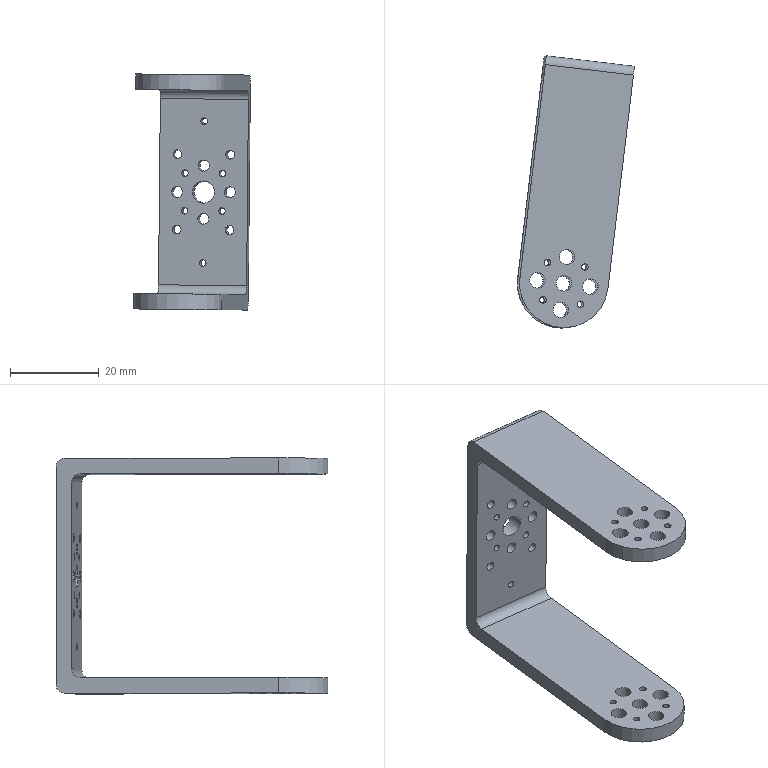Component | SolidWorks | Bracket3-1 | 1 solid | 83 faces | box 26.4 x 61.33 x 53.25 mm | volume 10774 mm3 | cylinder 74 | plane 9 | commonest cylinder face diameters 1.5 x28 3.5 x20 2 x8 2.5 x8 4 x4 5.94 x2 5 x2 20 x2 | material 45
build123d program:
from build123d import *

# Parameters (mm, degrees)
BOSS_EXTRUDE1_DEPTH    = 20
CUT_EXTRUDE1_DEPTH     = 87.499
SKETCH5_R              = 1.75
SKETCH5_R_2            = 0.75
CUT_EXTRUDE2_DEPTH     = 87.499
FILLET1_R              = 2
SKETCH6_R              = 2.5
SKETCH6_R_2            = 1.25
SKETCH6_R_3            = 0.75
CUT_EXTRUDE3_DEPTH     = 20
SKETCH7_R              = 1
CUT_EXTRUDE4_DEPTH     = 20
SKETCH8_R              = 0.75
CUT_EXTRUDE5_DEPTH     = 20
FILLET2_R              = 2
SKETCH1_R              = 2.97
SEAT_SERVOSPLINE_DEPTH = 0.6


with BuildPart() as part:
    # Sketch2 → Boss-Extrude1 (new body)
    with BuildSketch(Plane.XY):
        Polygon((4.869, 24.846), (4.869, 28.346), (65.369, 28.346), (65.369, -24.654), (4.869, -24.654), (4.869, -21.154), (61.869, -21.154), (61.869, 24.846), align=None)
    extrude(amount=-BOSS_EXTRUDE1_DEPTH)

    # Sketch3 → Cut-Extrude1 (cut, through all)
    with BuildSketch(Plane(origin=(0, 28.346, 0), x_dir=(1, 0, 0), z_dir=(0, 1, 0))):
        with BuildLine():
            ThreePointArc((14.869, 0), (7.798, 2.929), (4.869, 10))
            Line((4.869, 10), (4.869, 0))
            Line((4.869, 0), (14.869, 0))
        make_face()
        with BuildLine():
            ThreePointArc((4.869, 10), (7.798, 17.071), (14.869, 20))
            Line((14.869, 20), (4.869, 20))
            Line((4.869, 20), (4.869, 10))
        make_face()
    extrude(amount=-CUT_EXTRUDE1_DEPTH, mode=Mode.SUBTRACT)

    # Sketch5 → Cut-Extrude2 (cut, through all)
    with BuildSketch(Plane(origin=(0, 28.346, 0), x_dir=(1, 0, 0), z_dir=(0, 1, 0))):
        with Locations(Location((14.869, 10, 0), (0, 0, 270))):
            Circle(SKETCH5_R)
        with Locations(Location((20.869, 10, 0), (0, 0, 270))):
            Circle(SKETCH5_R)
        with Locations(Location((14.869, 4, 0), (0, 0, 270))):
            Circle(SKETCH5_R)
        with Locations(Location((8.869, 10, 0), (0, 0, 270))):
            Circle(SKETCH5_R)
        with Locations(Location((14.869, 16, 0), (0, 0, 270))):
            Circle(SKETCH5_R)
        with Locations(Location((19.112, 5.757, 0), (0, 0, 270))):
            Circle(SKETCH5_R_2)
        with Locations(Location((10.626, 5.757, 0), (0, 0, 270))):
            Circle(SKETCH5_R_2)
        with Locations(Location((10.626, 14.243, 0), (0, 0, 270))):
            Circle(SKETCH5_R_2)
        with Locations(Location((19.112, 14.243, 0), (0, 0, 270))):
            Circle(SKETCH5_R_2)
    extrude(amount=-CUT_EXTRUDE2_DEPTH, mode=Mode.SUBTRACT)

    # Fillet1
    fillet1_edges = [part.edges().sort_by_distance(p)[0] for p in [
        (65.369, 28.346, -10),
        (65.369, -24.654, -10),
    ]]
    fillet(fillet1_edges, radius=FILLET1_R)

    # Sketch6 → Cut-Extrude3 (cut)
    with BuildSketch(Plane(origin=(65.369, 0, 0), x_dir=(0, 0, -1), z_dir=(1, 0, 0))):
        with Locations((10, 1.846)):
            Circle(SKETCH6_R)
        with Locations((10, 7.846)):
            Circle(SKETCH6_R_2)
        with Locations((16, 1.846)):
            Circle(SKETCH6_R_2)
        with Locations((10, -4.154)):
            Circle(SKETCH6_R_2)
        with Locations((4, 1.846)):
            Circle(SKETCH6_R_2)
        with Locations((14.243, 6.089)):
            Circle(SKETCH6_R_3)
        with Locations((14.243, -2.397)):
            Circle(SKETCH6_R_3)
        with Locations((5.757, -2.397)):
            Circle(SKETCH6_R_3)
        with Locations((5.757, 6.089)):
            Circle(SKETCH6_R_3)
    extrude(amount=-CUT_EXTRUDE3_DEPTH, mode=Mode.SUBTRACT)

    # Sketch7 → Cut-Extrude4 (cut)
    with BuildSketch(Plane(origin=(65.369, 0, 0), x_dir=(0, 0, -1), z_dir=(1, 0, 0))):
        with Locations((16, 10.346)):
            Circle(SKETCH7_R)
        with Locations((4, 10.346)):
            Circle(SKETCH7_R)
        with Locations((4, -6.654)):
            Circle(SKETCH7_R)
        with Locations((16, -6.654)):
            Circle(SKETCH7_R)
    extrude(amount=-CUT_EXTRUDE4_DEPTH, mode=Mode.SUBTRACT)

    # Sketch8 → Cut-Extrude5 (cut)
    with BuildSketch(Plane(origin=(65.369, 0, 0), x_dir=(0, 0, -1), z_dir=(1, 0, 0))):
        with Locations((10, 17.846)):
            Circle(SKETCH8_R)
        with Locations((10, -14.154)):
            Circle(SKETCH8_R)
    extrude(amount=-CUT_EXTRUDE5_DEPTH, mode=Mode.SUBTRACT)

    # Fillet2
    fillet2_edges = [part.edges().sort_by_distance(p)[0] for p in [
        (61.869, -21.154, -10),
        (61.869, 24.846, -10),
    ]]
    fillet(fillet2_edges, radius=FILLET2_R)

    # Sketch1 → Seat-ServoSpline (cut)
    with BuildSketch(Plane(origin=(0, -21.154, 0), x_dir=(1, 0, 0), z_dir=(0, 1, 0))):
        with Locations(Location((14.869, 10, 0), (0, 0, 270))):
            Circle(SKETCH1_R)
    extrude(amount=-SEAT_SERVOSPLINE_DEPTH, mode=Mode.SUBTRACT)


solid = part.part

# Placed as in the assembly
solid = solid.moved(Location((-16.218, 16.912, 0.1588), (-85.302, -83.182, 4.732)))